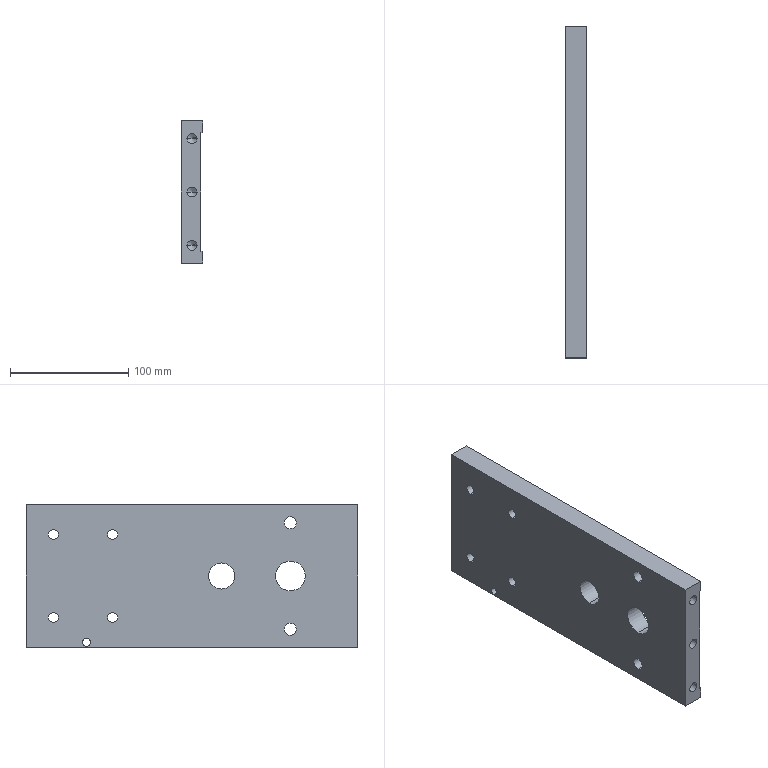Component | SolidWorks | ZL-11-02SmallUprightPlate-1 | 1 solid | 42 faces | box 18 x 280 x 120 mm | volume 537074 mm3 | cylinder 24 | plane 12 | cone 6 | commonest cylinder face diameters 8.5 x14 10.2 x4 6.5 x2 22 x2 25 x2
build123d program:
from build123d import *

# Parameters (mm, degrees)
EXTRUDE1_DEPTH            = 280
LPATTERN1_COUNT           = 3
LPATTERN1_PITCH           = 45
SKETCH4_R                 = 12.5
CUT_EXTRUDE1_DEPTH        = 287.831
SKETCH5_W                 = 5.1
SKETCH5_H                 = 16.5
SKETCH7_R                 = 11
CUT_EXTRUDE2_DEPTH        = 287.831
SKETCH8_R                 = 4.25
CUT_EXTRUDE3_DEPTH        = 287.831
LPATTERN2_COUNT           = 2
LPATTERN2_PITCH           = 50
LPATTERN2_COPY_1_SKETCH_R = 4.25
LPATTERN2_COPY_1_DEPTH    = 287.831
SKETCH9_R                 = 3.25
CUT_EXTRUDE4_DEPTH        = 287.922


with BuildPart() as part:
    # Sketch1 → Extrude1 (new body)
    with BuildSketch(Plane(origin=(0, 0, 0), x_dir=(1, 0, 0), z_dir=(0, 1, 0))):
        Polygon((-60, 0), (60, 0), (60, 18), (50, 18), (50, 16.5), (-50, 16.5), (-50, 18), (-60, 18), align=None)
    extrude(amount=-EXTRUDE1_DEPTH)

    # Sketch2 → M10 Tapped Hole1 (revolve, cut)
    with BuildSketch(Plane(origin=(-45, 0, -9), x_dir=(0, 0, 1), z_dir=(1, 0, 0))):
        Polygon((0, 0), (0, 27.054), (4.25, 24.5), (4.25, 0), align=None)
    m10_tapped_hole1 = revolve(axis=Axis((-45, 6.35, -9), (0, -1, 0)), mode=Mode.SUBTRACT)

    # LPattern1: M10 Tapped Hole1 ×3
    with Locations(*[(i * LPATTERN1_PITCH, 0, 0) for i in range(1, LPATTERN1_COUNT)]):
        add(m10_tapped_hole1, mode=Mode.SUBTRACT)

    # Sketch4 → Cut-Extrude1 (cut, through all)
    with BuildSketch(Plane(origin=(0, 0, -16.5), x_dir=(-1, 0, 0), z_dir=(0, 0, -1))):
        with Locations((0, -57)):
            Circle(SKETCH4_R)
    extrude(amount=-CUT_EXTRUDE1_DEPTH, mode=Mode.SUBTRACT)

    # Sketch5 → M12 Tapped Hole1 (revolve, cut)
    with BuildSketch(Plane(origin=(45, -57, -16.5), x_dir=(0, 1, 0), z_dir=(1, 0, 0))):
        with Locations((2.55, 8.25)):
            Rectangle(SKETCH5_W, SKETCH5_H)
    m12_tapped_hole1 = revolve(axis=Axis((45, -57, -22.85), (0, 0, 1)), mode=Mode.SUBTRACT)

    # Mirror1: M12 Tapped Hole1 across plane
    add(m12_tapped_hole1.mirror(Plane(origin=(0, 0, 0), x_dir=(0, 0, 1), z_dir=(1, 0, 0))), mode=Mode.SUBTRACT)

    # Sketch7 → Cut-Extrude2 (cut, through all)
    with BuildSketch(Plane(origin=(0, 0, -16.5), x_dir=(-1, 0, 0), z_dir=(0, 0, -1))):
        with Locations((0, -115)):
            Circle(SKETCH7_R)
    extrude(amount=-CUT_EXTRUDE2_DEPTH, mode=Mode.SUBTRACT)

    # Sketch8 → Cut-Extrude3 (cut, through all)
    with BuildSketch(Plane(origin=(0, 0, -16.5), x_dir=(-1, 0, 0), z_dir=(0, 0, -1))):
        with Locations((-35, -207)):
            Circle(SKETCH8_R)
    cut_extrude3 = extrude(amount=-CUT_EXTRUDE3_DEPTH, mode=Mode.SUBTRACT)

    # Mirror2: Cut-Extrude3 across plane
    add(cut_extrude3.mirror(Plane(origin=(0, 0, 0), x_dir=(0, 0, 1), z_dir=(1, 0, 0))), mode=Mode.SUBTRACT)

    # LPattern2: Cut-Extrude3 ×2
    with Locations(*[(0, -i * LPATTERN2_PITCH, 0) for i in range(1, LPATTERN2_COUNT)]):
        add(cut_extrude3, mode=Mode.SUBTRACT)

    # LPattern2 copy 1 sketch → LPattern2 copy 1 (cut, through all)
    with BuildSketch(Plane(origin=(0, -50, -16.5), x_dir=(1, 0, 0), z_dir=(0, 0, -1))):
        with Locations((-35, 207)):
            Circle(LPATTERN2_COPY_1_SKETCH_R)
    extrude(amount=-LPATTERN2_COPY_1_DEPTH, mode=Mode.SUBTRACT)

    # Sketch9 → Cut-Extrude4 (cut, through all)
    with BuildSketch(Plane(origin=(0, 0, -18), x_dir=(-1, 0, 0), z_dir=(0, 0, -1))):
        with Locations((-56, -229)):
            Circle(SKETCH9_R)
    extrude(amount=-CUT_EXTRUDE4_DEPTH, mode=Mode.SUBTRACT)


solid = part.part

# Placed as in the assembly
solid = solid.moved(Location((-186.448, 54.22, 0), (180, -90, 0)))